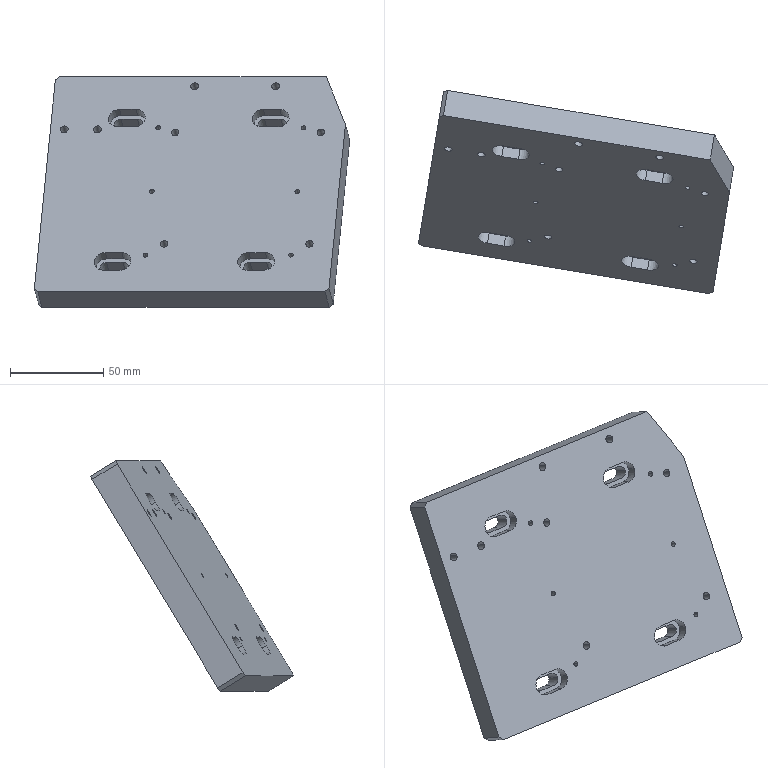Component | SolidWorks | 14AC-24-1-012-1 | 1 solid | 102 faces | box 168.9 x 108.62 x 123.49 mm | volume 332079 mm3 | cylinder 52 | plane 30 | cone 20 | commonest cylinder face diameters 6.6 x12 11 x12 2.5 x12 4 x8 4.2 x8
build123d program:
from build123d import *

# Parameters (mm, degrees)
SKETCH1_W                                       = 160
SKETCH1_H                                       = 135
BOSS_EXTRUDE1_DEPTH                             = 16
M5_TAPPED_HOLE1_D                               = 4.2
M5_TAPPED_HOLE1_DEPTH                           = 12.4
M5_TAPPED_HOLE1_TIP                             = 1.262
M5_TAPPED_HOLE2_D                               = 4.2
M5_TAPPED_HOLE2_DEPTH                           = 12.4
M5_TAPPED_HOLE2_TIP                             = 1.262
M6_HEX_SOCKET_HEAD_CAP_SCREW_CBORE1_D           = 6.6
M6_HEX_SOCKET_HEAD_CAP_SCREW_CBORE1_CBORE_D     = 11
M6_HEX_SOCKET_HEAD_CAP_SCREW_CBORE1_CBORE_DEPTH = 6.4
CHAMFER1_SIZE                                   = 2
M3_TAPPED_HOLE2_AT_2_COUNT                      = 2
M3_TAPPED_HOLE2_AT_2_PITCH                      = 40
M3_TAPPED_HOLE2_AT_3_COUNT                      = 2
M3_TAPPED_HOLE2_AT_3_PITCH                      = 80
LPATTERN2_COUNT                                 = 2
LPATTERN2_PITCH                                 = 79
SKETCH14_R                                      = 2
CUT_EXTRUDE6_DEPTH                              = 106.888
LPATTERN3_COUNT                                 = 2
LPATTERN3_PITCH                                 = 79
CUT_EXTRUDE7_DEPTH                              = 6.4
CUT_EXTRUDE8_DEPTH                              = 106.111
LPATTERN4_COUNT                                 = 2
LPATTERN4_PITCH                                 = 90
LPATTERN4_COUNT_DIR2                            = 2
LPATTERN4_PITCH_DIR2                            = 78
CHAMFER2_SIZE                                   = 30
CHAMFER2_SIZE2                                  = 13


with BuildPart() as part:
    # Sketch1 → Boss-Extrude1 (new body)
    with BuildSketch(Plane.XY):
        Rectangle(SKETCH1_W, SKETCH1_H)
    extrude(amount=BOSS_EXTRUDE1_DEPTH)

    # M5 Tapped Hole1
    with Locations(Plane(origin=(-4, 61.5, 16), x_dir=(1, 0, 0), z_dir=(0, 0, 1))):
        with Locations((0, 0), (44, 0)):
            Hole(M5_TAPPED_HOLE1_D / 2, depth=M5_TAPPED_HOLE1_DEPTH)
            with Locations((0, 0, -(M5_TAPPED_HOLE1_DEPTH + M5_TAPPED_HOLE1_TIP / 2))):  # 118° drill point
                Cone(0, M5_TAPPED_HOLE1_D / 2, M5_TAPPED_HOLE1_TIP, mode=Mode.SUBTRACT)

    # M5 Tapped Hole2
    with Locations(Plane(origin=(-72.5, 34.5, 16), x_dir=(1, 0, 0), z_dir=(0, 0, 1))):
        with Locations((0, 0), (18, 0)):
            Hole(M5_TAPPED_HOLE2_D / 2, depth=M5_TAPPED_HOLE2_DEPTH)
            with Locations((0, 0, -(M5_TAPPED_HOLE2_DEPTH + M5_TAPPED_HOLE2_TIP / 2))):  # 118° drill point
                Cone(0, M5_TAPPED_HOLE2_D / 2, M5_TAPPED_HOLE2_TIP, mode=Mode.SUBTRACT)

    # M6 Hex Socket Head Cap Screw CBORE1 (through all)
    with Locations(Plane(origin=(-39, 41.5, 16), x_dir=(1, 0, 0), z_dir=(0, 0, 1))):
        with Locations((0, 0), (78, 0), (0, -90), (78, -90)):
            CounterBoreHole(M6_HEX_SOCKET_HEAD_CAP_SCREW_CBORE1_D / 2, M6_HEX_SOCKET_HEAD_CAP_SCREW_CBORE1_CBORE_D / 2, M6_HEX_SOCKET_HEAD_CAP_SCREW_CBORE1_CBORE_DEPTH)

    # Chamfer1
    chamfer1_edges = [part.edges().sort_by_distance(p)[0] for p in [
        (80, -67.5, 8),
        (-80, -67.5, 8),
        (-80, 67.5, 8),
    ]]
    chamfer(chamfer1_edges, length=CHAMFER1_SIZE)

    # Sketch12 → M3 Tapped Hole2 (revolve, cut)
    with BuildSketch(Plane(origin=(57.5, 35.5, 16), x_dir=(0, -1, 0), z_dir=(1, 0, 0))):
        Polygon((0, 0), (0, 8.251), (1.25, 7.5), (1.25, 0), align=None)
    m3_tapped_hole2 = revolve(axis=Axis((57.5, 35.5, 22.35), (0, 0, -1)), mode=Mode.SUBTRACT)

    # M3 Tapped Hole2 at 2: M3 Tapped Hole2 ×2
    with Locations(*[(0, -i * M3_TAPPED_HOLE2_AT_2_PITCH, 0) for i in range(1, M3_TAPPED_HOLE2_AT_2_COUNT)]):
        add(m3_tapped_hole2, mode=Mode.SUBTRACT)

    # M3 Tapped Hole2 at 3: M3 Tapped Hole2 ×2
    with Locations(*[(0, -i * M3_TAPPED_HOLE2_AT_3_PITCH, 0) for i in range(1, M3_TAPPED_HOLE2_AT_3_COUNT)]):
        add(m3_tapped_hole2, mode=Mode.SUBTRACT)

    # LPattern2: M3 Tapped Hole2 ×2
    with Locations(*[(-i * LPATTERN2_PITCH, 0, 0) for i in range(1, LPATTERN2_COUNT)]):
        add(m3_tapped_hole2, mode=Mode.SUBTRACT)

    # LPattern2 copy 1 sketch → LPattern2 copy 1 (revolve, cut)
    with BuildSketch(Plane(origin=(-21.5, -4.5, 16), x_dir=(0, -1, 0), z_dir=(1, 0, 0))):
        Polygon((0, 0), (0, 8.251), (1.25, 7.5), (1.25, 0), align=None)
    revolve(axis=Axis((-21.5, -4.5, 22.35), (0, 0, -1)), mode=Mode.SUBTRACT)

    # LPattern2 copy 2 sketch → LPattern2 copy 2 (revolve, cut)
    with BuildSketch(Plane(origin=(-21.5, -44.5, 16), x_dir=(0, -1, 0), z_dir=(1, 0, 0))):
        Polygon((0, 0), (0, 8.251), (1.25, 7.5), (1.25, 0), align=None)
    revolve(axis=Axis((-21.5, -44.5, 22.35), (0, 0, -1)), mode=Mode.SUBTRACT)

    # Sketch14 → Cut-Extrude6 (cut, through all)
    with BuildSketch(Plane.XY.offset(16)):
        with Locations((67, 32.5)):
            Circle(SKETCH14_R)
        with Locations((67, -37.5)):
            Circle(SKETCH14_R)
    cut_extrude6 = extrude(amount=-CUT_EXTRUDE6_DEPTH, mode=Mode.SUBTRACT)

    # LPattern3: Cut-Extrude6 ×2
    with Locations(*[(-i * LPATTERN3_PITCH, 0, 0) for i in range(1, LPATTERN3_COUNT)]):
        add(cut_extrude6, mode=Mode.SUBTRACT)

    # Sketch15 → Cut-Extrude7 (cut)
    with BuildSketch(Plane.XY.offset(16)):
        with BuildLine():
            Line((-43.5, -43), (-34.5, -43))
            ThreePointArc((-34.5, -43), (-29, -48.5), (-34.5, -54))
            Line((-34.5, -54), (-43.5, -54))
            ThreePointArc((-43.5, -54), (-49, -48.5), (-43.5, -43))
        make_face()
    cut_extrude7 = extrude(amount=-CUT_EXTRUDE7_DEPTH, mode=Mode.SUBTRACT)

    # Sketch16 → Cut-Extrude8 (cut, through all)
    with BuildSketch(Plane.XY.offset(9.6)):
        with BuildLine():
            Line((-43.5, -45.2), (-34.5, -45.2))
            ThreePointArc((-34.5, -45.2), (-31.2, -48.5), (-34.5, -51.8))
            Line((-34.5, -51.8), (-43.5, -51.8))
            ThreePointArc((-43.5, -51.8), (-46.8, -48.5), (-43.5, -45.2))
        make_face()
    cut_extrude8 = extrude(amount=-CUT_EXTRUDE8_DEPTH, mode=Mode.SUBTRACT)

    # LPattern4: Cut-Extrude7, Cut-Extrude8 2 × 2
    with Locations(*[(j * LPATTERN4_PITCH_DIR2, i * LPATTERN4_PITCH, 0) for i in range(LPATTERN4_COUNT) for j in range(LPATTERN4_COUNT_DIR2) if (i, j) != (0, 0)]):
        add(cut_extrude7, mode=Mode.SUBTRACT)
        add(cut_extrude8, mode=Mode.SUBTRACT)

    # Chamfer2
    chamfer2_edges = [part.edges().sort_by_distance(p)[0] for p in [
        (80, 67.5, 8),
    ]]
    chamfer2_side = [part.faces().sort_by_distance(p)[0] for p in [
        (80, 1, 8),
    ]]
    chamfer(chamfer2_edges, length=CHAMFER2_SIZE, length2=CHAMFER2_SIZE2, reference=chamfer2_side[0])


solid = part.part

# Placed as in the assembly
solid = solid.moved(Location((396.998, -118.853, -202.414), (58.173, -8.052, -4.969)))